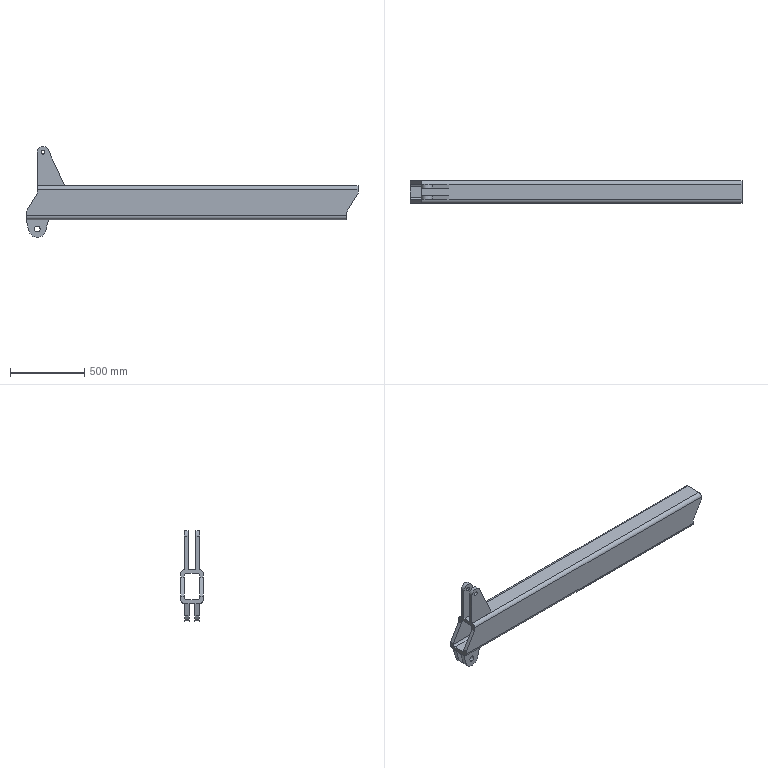Component | NX | ARM_SECTION_4 | 1 solid | 46 faces | volume 37931502 mm3 | plane 30 | cylinder 16 | commonest cylinder face diameters 50 x4 32 x4 76.2 x2 25.4 x2 114.3 x2 38.1 x2